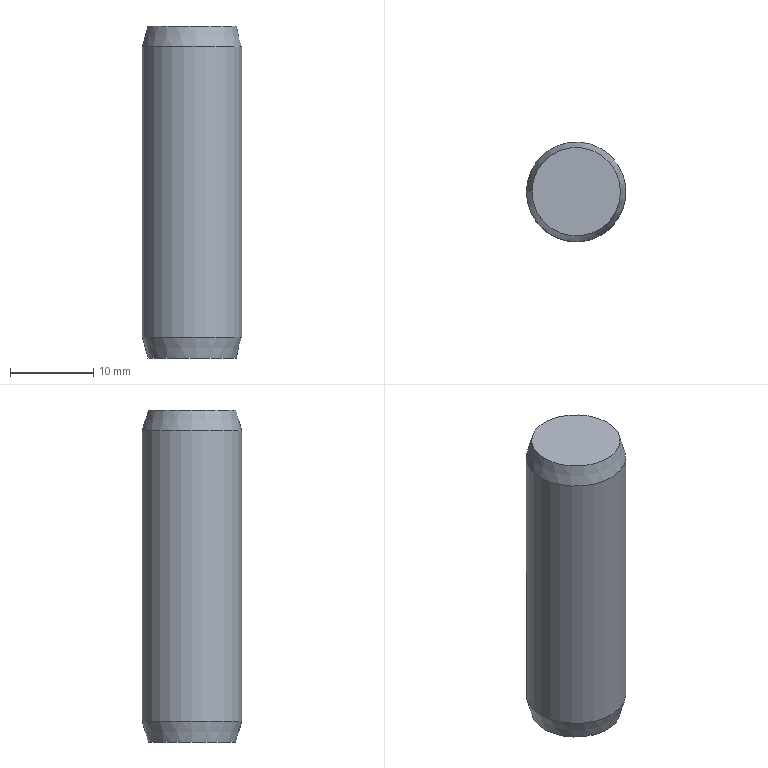Component | NX | GB-T119_1-2000_12X40_2 | 1 solid | 5 faces | box 12 x 12 x 40 mm | volume 4463 mm3 | plane 2 | cone 2 | cylinder 1 | commonest cylinder face diameters 12 x1
STEP:
#1=CARTESIAN_POINT('',(0.,0.,0.));
#2=DIRECTION('',(0.,0.,1.));
#3=DIRECTION('',(1.,0.,0.));
#4=AXIS2_PLACEMENT_3D('',#1,#2,#3);
#5=CARTESIAN_POINT('',(-137.33,-80.,160.));
#6=VERTEX_POINT('',#5);
#7=CARTESIAN_POINT('',(-132.,-80.,160.));
#8=DIRECTION('',(0.,0.,-1.));
#9=DIRECTION('',(-1.,0.,0.));
#10=AXIS2_PLACEMENT_3D('',#7,#8,#9);
#11=CIRCLE('',#10,5.33);
#12=CARTESIAN_POINT('',(-132.,-80.,160.));
#13=DIRECTION('',(0.,0.,-1.));
#14=DIRECTION('',(-1.,0.,0.));
#15=AXIS2_PLACEMENT_3D('',#12,#13,#14);
#16=PLANE('',#15);
#17=CARTESIAN_POINT('',(0.,0.));
#18=DIRECTION('',(1.,0.));
#19=AXIS2_PLACEMENT_2D('',#17,#18);
#20=CIRCLE('',#19,5.33);
#21=(GEOMETRIC_REPRESENTATION_CONTEXT(2)PARAMETRIC_REPRESENTATION_CONTEXT()REPRESENTATION_CONTEXT('',''));
#22=DEFINITIONAL_REPRESENTATION('',(#20),#21);
#23=PCURVE('',#16,#22);
#24=CARTESIAN_POINT('',(-132.,-80.,160.));
#25=DIRECTION('',(0.,0.,1.));
#26=DIRECTION('',(1.,0.,0.));
#27=AXIS2_PLACEMENT_3D('',#24,#25,#26);
#28=CONICAL_SURFACE('',#27,5.33,0.2618);
#29=CARTESIAN_POINT('',(9.425,0.));
#30=DIRECTION('',(-1.,0.));
#31=VECTOR('',#30,1.);
#32=LINE('',#29,#31);
#33=(GEOMETRIC_REPRESENTATION_CONTEXT(2)PARAMETRIC_REPRESENTATION_CONTEXT()REPRESENTATION_CONTEXT('',''));
#34=DEFINITIONAL_REPRESENTATION('',(#32),#33);
#35=PCURVE('',#28,#34);
#36=SURFACE_CURVE('',#11,(#23,#35),.PCURVE_S1.);
#37=EDGE_CURVE('',#6,#6,#36,.T.);
#38=ORIENTED_EDGE('',*,*,#37,.T.);
#39=EDGE_LOOP('',(#38));
#40=FACE_BOUND('',#39,.T.);
#41=ADVANCED_FACE('',(#40),#16,.T.);
#42=CARTESIAN_POINT('',(-138.,-80.,162.5));
#43=VERTEX_POINT('',#42);
#44=CARTESIAN_POINT('',(-132.,-80.,162.5));
#45=DIRECTION('',(0.,0.,-1.));
#46=DIRECTION('',(-1.,0.,0.));
#47=AXIS2_PLACEMENT_3D('',#44,#45,#46);
#48=CIRCLE('',#47,6.);
#49=CARTESIAN_POINT('',(9.425,2.5));
#50=DIRECTION('',(-1.,0.));
#51=VECTOR('',#50,1.);
#52=LINE('',#49,#51);
#53=(GEOMETRIC_REPRESENTATION_CONTEXT(2)PARAMETRIC_REPRESENTATION_CONTEXT()REPRESENTATION_CONTEXT('',''));
#54=DEFINITIONAL_REPRESENTATION('',(#52),#53);
#55=PCURVE('',#28,#54);
#56=CARTESIAN_POINT('',(-132.,-80.,200.));
#57=DIRECTION('',(0.,0.,-1.));
#58=DIRECTION('',(-1.,0.,0.));
#59=AXIS2_PLACEMENT_3D('',#56,#57,#58);
#60=CYLINDRICAL_SURFACE('',#59,6.);
#61=CARTESIAN_POINT('',(0.,37.5));
#62=DIRECTION('',(1.,0.));
#63=VECTOR('',#62,1.);
#64=LINE('',#61,#63);
#65=(GEOMETRIC_REPRESENTATION_CONTEXT(2)PARAMETRIC_REPRESENTATION_CONTEXT()REPRESENTATION_CONTEXT('',''));
#66=DEFINITIONAL_REPRESENTATION('',(#64),#65);
#67=PCURVE('',#60,#66);
#68=SURFACE_CURVE('',#48,(#55,#67),.PCURVE_S1.);
#69=EDGE_CURVE('',#43,#43,#68,.T.);
#70=ORIENTED_EDGE('',*,*,#69,.T.);
#71=CARTESIAN_POINT('',(-137.33,-80.,160.));
#72=CARTESIAN_POINT('',(-138.,-80.,162.5));
#73=B_SPLINE_CURVE_WITH_KNOTS('',1,(#71,#72),.UNSPECIFIED.,.F.,.F.,(2,2),(0.,2.588),.PIECEWISE_BEZIER_KNOTS.);
#74=CARTESIAN_POINT('',(3.142,0.));
#75=DIRECTION('',(0.,1.));
#76=VECTOR('',#75,1.);
#77=LINE('',#74,#76);
#78=(GEOMETRIC_REPRESENTATION_CONTEXT(2)PARAMETRIC_REPRESENTATION_CONTEXT()REPRESENTATION_CONTEXT('',''));
#79=DEFINITIONAL_REPRESENTATION('',(#77),#78);
#80=PCURVE('',#28,#79);
#81=CARTESIAN_POINT('',(9.425,0.));
#82=DIRECTION('',(0.,1.));
#83=VECTOR('',#82,1.);
#84=LINE('',#81,#83);
#85=(GEOMETRIC_REPRESENTATION_CONTEXT(2)PARAMETRIC_REPRESENTATION_CONTEXT()REPRESENTATION_CONTEXT('',''));
#86=DEFINITIONAL_REPRESENTATION('',(#84),#85);
#87=PCURVE('',#28,#86);
#88=SEAM_CURVE('',#73,(#80,#87),.PCURVE_S1.);
#89=EDGE_CURVE('',#6,#43,#88,.T.);
#90=ORIENTED_EDGE('',*,*,#89,.F.);
#91=ORIENTED_EDGE('',*,*,#37,.F.);
#92=ORIENTED_EDGE('',*,*,#89,.T.);
#93=EDGE_LOOP('',(#70,#90,#91,#92));
#94=FACE_BOUND('',#93,.T.);
#95=ADVANCED_FACE('',(#94),#28,.T.);
#96=CARTESIAN_POINT('',(-138.,-80.,197.5));
#97=VERTEX_POINT('',#96);
#98=CARTESIAN_POINT('',(-132.,-80.,197.5));
#99=DIRECTION('',(0.,0.,-1.));
#100=DIRECTION('',(-1.,0.,0.));
#101=AXIS2_PLACEMENT_3D('',#98,#99,#100);
#102=CIRCLE('',#101,6.);
#103=CARTESIAN_POINT('',(0.,2.5));
#104=DIRECTION('',(1.,0.));
#105=VECTOR('',#104,1.);
#106=LINE('',#103,#105);
#107=(GEOMETRIC_REPRESENTATION_CONTEXT(2)PARAMETRIC_REPRESENTATION_CONTEXT()REPRESENTATION_CONTEXT('',''));
#108=DEFINITIONAL_REPRESENTATION('',(#106),#107);
#109=PCURVE('',#60,#108);
#110=CARTESIAN_POINT('',(-132.,-80.,197.5));
#111=DIRECTION('',(0.,0.,-1.));
#112=DIRECTION('',(-1.,0.,0.));
#113=AXIS2_PLACEMENT_3D('',#110,#111,#112);
#114=CONICAL_SURFACE('',#113,6.,0.2618);
#115=CARTESIAN_POINT('',(0.,-0.));
#116=DIRECTION('',(1.,0.));
#117=VECTOR('',#116,1.);
#118=LINE('',#115,#117);
#119=(GEOMETRIC_REPRESENTATION_CONTEXT(2)PARAMETRIC_REPRESENTATION_CONTEXT()REPRESENTATION_CONTEXT('',''));
#120=DEFINITIONAL_REPRESENTATION('',(#118),#119);
#121=PCURVE('',#114,#120);
#122=SURFACE_CURVE('',#102,(#109,#121),.PCURVE_S1.);
#123=EDGE_CURVE('',#97,#97,#122,.T.);
#124=ORIENTED_EDGE('',*,*,#123,.T.);
#125=CARTESIAN_POINT('',(-138.,-80.,197.5));
#126=CARTESIAN_POINT('',(-138.,-80.,162.5));
#127=B_SPLINE_CURVE_WITH_KNOTS('',1,(#125,#126),.UNSPECIFIED.,.F.,.F.,(2,2),(2.5,37.5),.PIECEWISE_BEZIER_KNOTS.);
#128=CARTESIAN_POINT('',(6.283,0.));
#129=DIRECTION('',(0.,1.));
#130=VECTOR('',#129,1.);
#131=LINE('',#128,#130);
#132=(GEOMETRIC_REPRESENTATION_CONTEXT(2)PARAMETRIC_REPRESENTATION_CONTEXT()REPRESENTATION_CONTEXT('',''));
#133=DEFINITIONAL_REPRESENTATION('',(#131),#132);
#134=PCURVE('',#60,#133);
#135=CARTESIAN_POINT('',(0.,0.));
#136=DIRECTION('',(0.,1.));
#137=VECTOR('',#136,1.);
#138=LINE('',#135,#137);
#139=(GEOMETRIC_REPRESENTATION_CONTEXT(2)PARAMETRIC_REPRESENTATION_CONTEXT()REPRESENTATION_CONTEXT('',''));
#140=DEFINITIONAL_REPRESENTATION('',(#138),#139);
#141=PCURVE('',#60,#140);
#142=SEAM_CURVE('',#127,(#134,#141),.PCURVE_S1.);
#143=EDGE_CURVE('',#97,#43,#142,.T.);
#144=ORIENTED_EDGE('',*,*,#143,.T.);
#145=ORIENTED_EDGE('',*,*,#69,.F.);
#146=ORIENTED_EDGE('',*,*,#143,.F.);
#147=EDGE_LOOP('',(#124,#144,#145,#146));
#148=FACE_BOUND('',#147,.T.);
#149=ADVANCED_FACE('',(#148),#60,.T.);
#150=CARTESIAN_POINT('',(-137.33,-80.,200.));
#151=VERTEX_POINT('',#150);
#152=CARTESIAN_POINT('',(-132.,-80.,200.));
#153=DIRECTION('',(0.,0.,-1.));
#154=DIRECTION('',(-1.,0.,0.));
#155=AXIS2_PLACEMENT_3D('',#152,#153,#154);
#156=CIRCLE('',#155,5.33);
#157=CARTESIAN_POINT('',(0.,-2.5));
#158=DIRECTION('',(1.,0.));
#159=VECTOR('',#158,1.);
#160=LINE('',#157,#159);
#161=(GEOMETRIC_REPRESENTATION_CONTEXT(2)PARAMETRIC_REPRESENTATION_CONTEXT()REPRESENTATION_CONTEXT('',''));
#162=DEFINITIONAL_REPRESENTATION('',(#160),#161);
#163=PCURVE('',#114,#162);
#164=CARTESIAN_POINT('',(-126.67,-80.,200.));
#165=DIRECTION('',(0.,0.,1.));
#166=DIRECTION('',(1.,0.,0.));
#167=AXIS2_PLACEMENT_3D('',#164,#165,#166);
#168=PLANE('',#167);
#169=CARTESIAN_POINT('',(-10.66,0.));
#170=CARTESIAN_POINT('',(-10.66,9.232));
#171=CARTESIAN_POINT('',(-2.665,4.616));
#172=CARTESIAN_POINT('',(5.33,0.));
#173=CARTESIAN_POINT('',(-2.665,-4.616));
#174=CARTESIAN_POINT('',(-10.66,-9.232));
#175=CARTESIAN_POINT('',(-10.66,0.));
#176=(BOUNDED_CURVE()B_SPLINE_CURVE(2,(#169,#170,#171,#172,#173,#174,#175),.UNSPECIFIED.,.T.,.F.)B_SPLINE_CURVE_WITH_KNOTS((1,2,2,2,2,1),(-2.094,0.,2.094,4.189,6.283,8.378),.UNSPECIFIED.)CURVE()GEOMETRIC_REPRESENTATION_ITEM()RATIONAL_B_SPLINE_CURVE((1.,0.5,1.,0.5,1.,0.5,1.))REPRESENTATION_ITEM(''));
#177=(GEOMETRIC_REPRESENTATION_CONTEXT(2)PARAMETRIC_REPRESENTATION_CONTEXT()REPRESENTATION_CONTEXT('',''));
#178=DEFINITIONAL_REPRESENTATION('',(#176),#177);
#179=PCURVE('',#168,#178);
#180=SURFACE_CURVE('',#156,(#163,#179),.PCURVE_S1.);
#181=EDGE_CURVE('',#151,#151,#180,.T.);
#182=ORIENTED_EDGE('',*,*,#181,.T.);
#183=CARTESIAN_POINT('',(-137.33,-80.,200.));
#184=CARTESIAN_POINT('',(-138.,-80.,197.5));
#185=B_SPLINE_CURVE_WITH_KNOTS('',1,(#183,#184),.UNSPECIFIED.,.F.,.F.,(2,2),(-2.588,-0.),.PIECEWISE_BEZIER_KNOTS.);
#186=CARTESIAN_POINT('',(6.283,0.));
#187=DIRECTION('',(0.,1.));
#188=VECTOR('',#187,1.);
#189=LINE('',#186,#188);
#190=(GEOMETRIC_REPRESENTATION_CONTEXT(2)PARAMETRIC_REPRESENTATION_CONTEXT()REPRESENTATION_CONTEXT('',''));
#191=DEFINITIONAL_REPRESENTATION('',(#189),#190);
#192=PCURVE('',#114,#191);
#193=CARTESIAN_POINT('',(0.,0.));
#194=DIRECTION('',(0.,1.));
#195=VECTOR('',#194,1.);
#196=LINE('',#193,#195);
#197=(GEOMETRIC_REPRESENTATION_CONTEXT(2)PARAMETRIC_REPRESENTATION_CONTEXT()REPRESENTATION_CONTEXT('',''));
#198=DEFINITIONAL_REPRESENTATION('',(#196),#197);
#199=PCURVE('',#114,#198);
#200=SEAM_CURVE('',#185,(#192,#199),.PCURVE_S1.);
#201=EDGE_CURVE('',#151,#97,#200,.T.);
#202=ORIENTED_EDGE('',*,*,#201,.T.);
#203=ORIENTED_EDGE('',*,*,#123,.F.);
#204=ORIENTED_EDGE('',*,*,#201,.F.);
#205=EDGE_LOOP('',(#182,#202,#203,#204));
#206=FACE_BOUND('',#205,.T.);
#207=ADVANCED_FACE('',(#206),#114,.T.);
#208=ORIENTED_EDGE('',*,*,#181,.F.);
#209=EDGE_LOOP('',(#208));
#210=FACE_BOUND('',#209,.T.);
#211=ADVANCED_FACE('',(#210),#168,.T.);
#212=CLOSED_SHELL('',(#41,#95,#149,#207,#211));
#213=MANIFOLD_SOLID_BREP('',#212);
#214=(LENGTH_UNIT()NAMED_UNIT(*)SI_UNIT(.MILLI.,.METRE.));
#215=UNCERTAINTY_MEASURE_WITH_UNIT(LENGTH_MEASURE(0.00001),#214,'','');
#216=(NAMED_UNIT(*)PLANE_ANGLE_UNIT()SI_UNIT($,.RADIAN.));
#217=(NAMED_UNIT(*)SI_UNIT($,.STERADIAN.)SOLID_ANGLE_UNIT());
#218=(GEOMETRIC_REPRESENTATION_CONTEXT(3)GLOBAL_UNCERTAINTY_ASSIGNED_CONTEXT((#215))GLOBAL_UNIT_ASSIGNED_CONTEXT((#214,#216,#217))REPRESENTATION_CONTEXT('',''));
#219=ADVANCED_BREP_SHAPE_REPRESENTATION('',(#4,#213),#218);